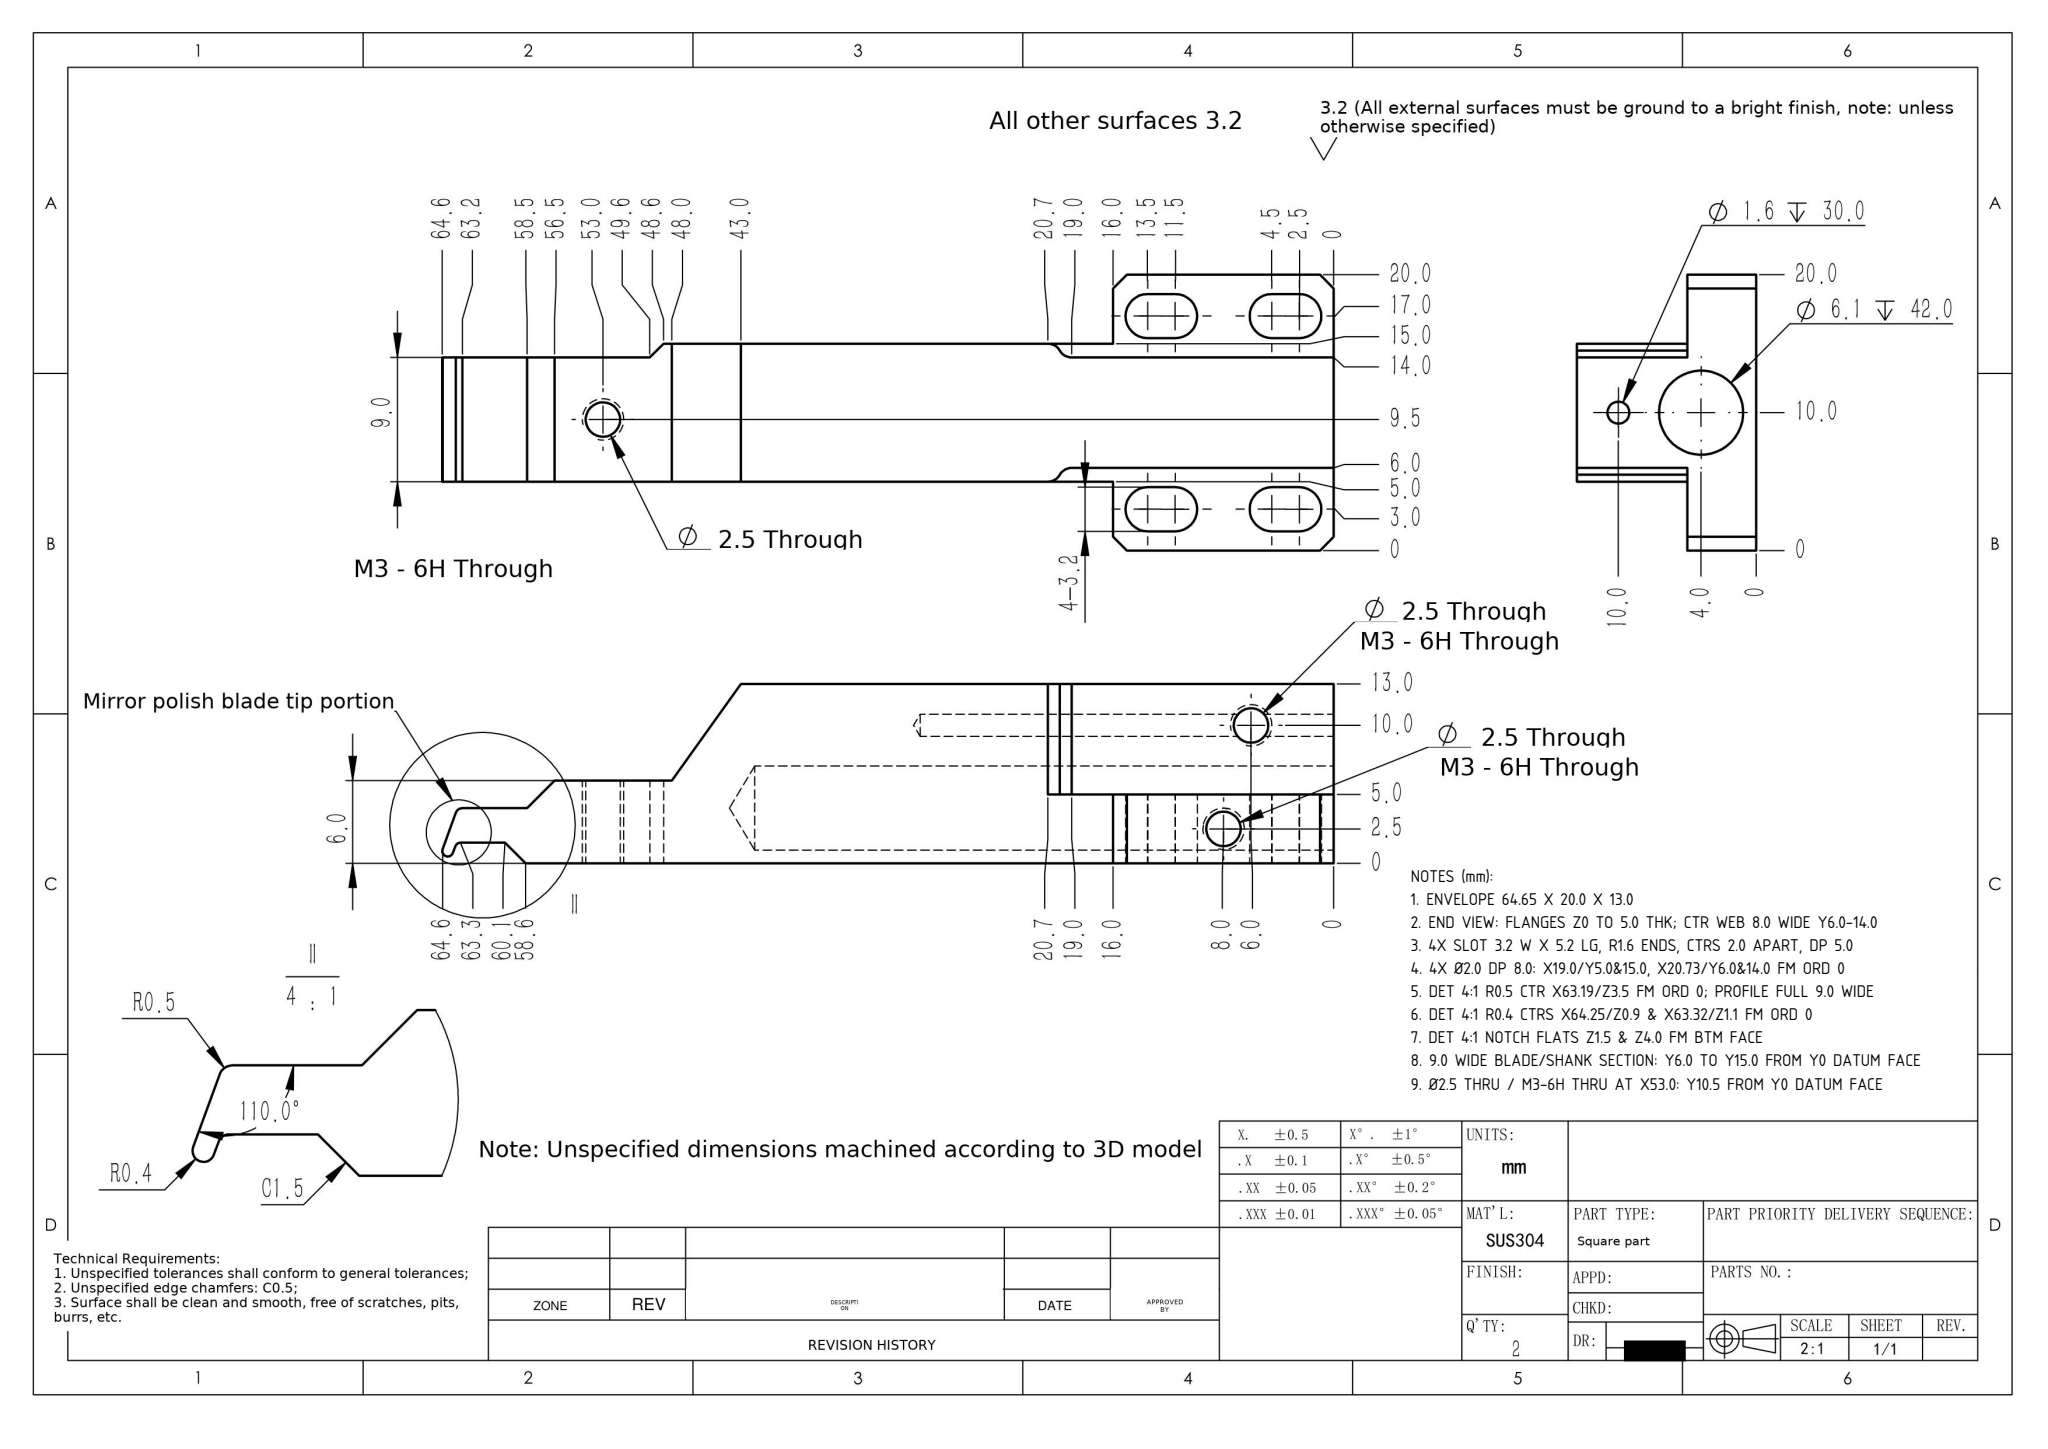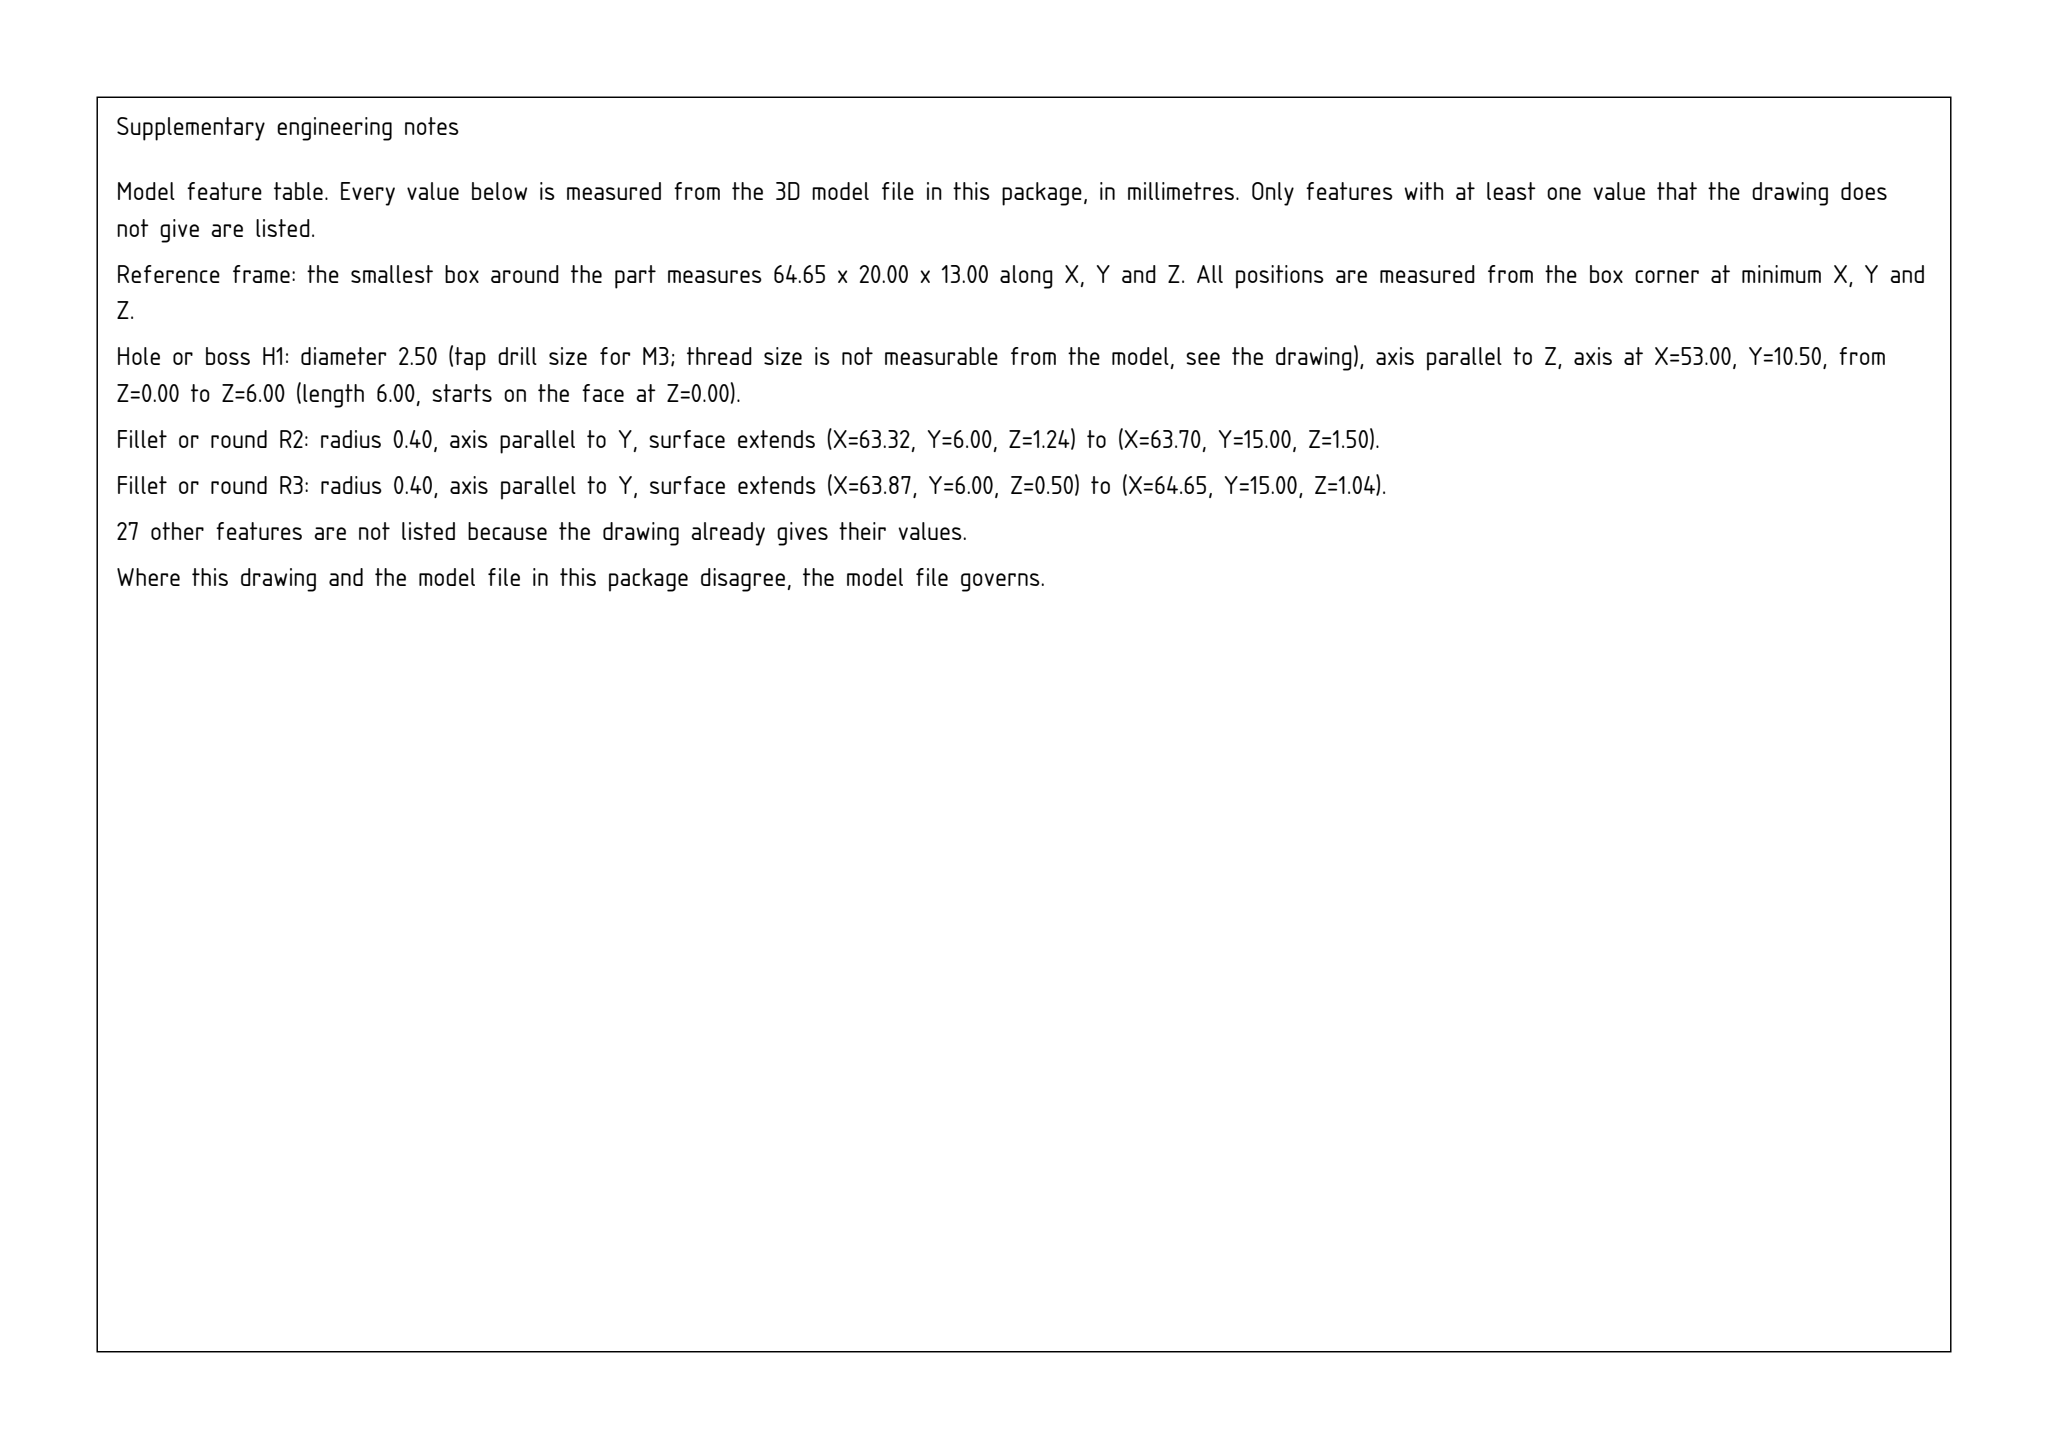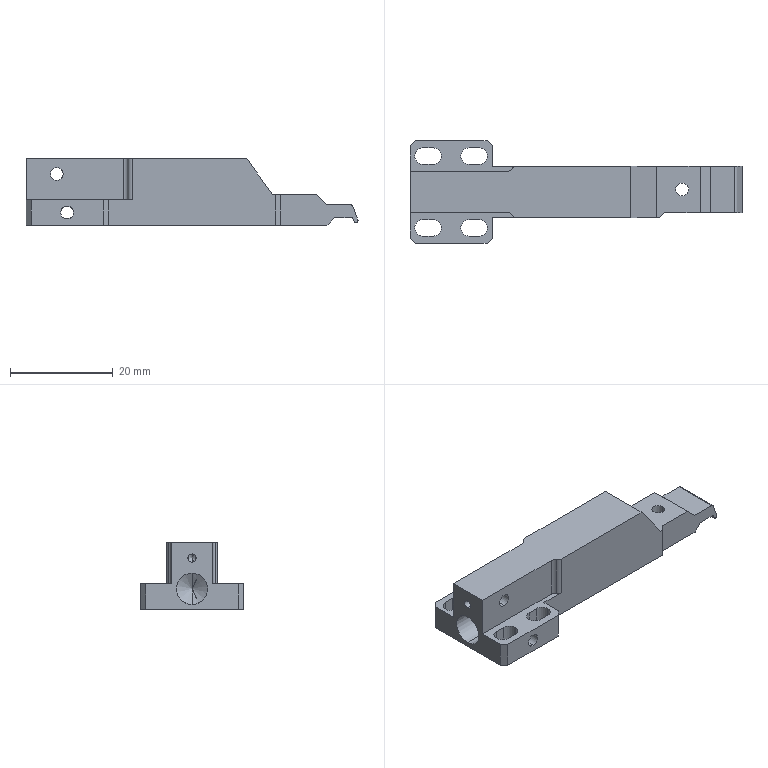Part | SolidWorks | mm | 1 solid | 74 faces | box 64.65 x 20 x 13 mm | volume 5503 mm3 | cylinder 35 | plane 35 | cone 4 | commonest cylinder face diameters 3.2 x12 2.5 x8 0.8 x4 1.6 x4 2 x4 6.1 x2 1 x1
Drawing notes:
ENVELOPE 64.65 X 20.0 X 13.0 | from the solid: bbox_xyz 64.646 x 20.0 x 13.0
END VIEW: FLANGES Z0 TO 5.0 THK; CTR WEB 8.0 WIDE Y6.0-14.0 | from the solid: z-planes 0/5.0; d2.5 y-hole len 8.0 betw y-planes 6.0 & 14.0
4X SLOT 3.2 W X 5.2 LG, R1.6 ENDS, CTRS 2.0 APART, DP 5.0 | from the solid: d3.2 z-cyls at x2.5/4.5 & x11.5/13.5, y3.0 & y17.0, len 5.0
4X Ø2.0 DP 8.0: X19.0/Y5.0&15.0, X20.73/Y6.0&14.0 FM ORD 0 | from the solid: dia 2.0 z-cyls len 8.0 at (19.0,5.0),(19.0,15.0),(20.73,6.0),(20.73,14.0)
DET 4:1 R0.5 CTR X63.19/Z3.5 FM ORD 0; PROFILE FULL 9.0 WIDE | from the solid: cyl d1.0 axis y at (63.19,z3.5), len 9.0 = shank width y5.0-14.0
DET 4:1 R0.4 CTRS X64.25/Z0.9 & X63.32/Z1.1 FM ORD 0 | from the solid: cyl d0.8 axis y at (63.32,z1.1) and (64.25,z0.9), len 9.0
DET 4:1 NOTCH FLATS Z1.5 & Z4.0 FM BTM FACE | from the solid: z-normal planes at 1.5 and 4.0 within blade tip zone
9.0 WIDE BLADE/SHANK SECTION: Y6.0 TO Y15.0 FROM Y0 DATUM FACE | from the solid: y planes at 6.0 and 15.0 bound the 9.0 band; bbox Y0-20.0
Ø2.5 THRU / M3-6H THRU AT X53.0: Y10.5 FROM Y0 DATUM FACE | from the solid: cylinder [2.5,'z',[53.0,10.5,null],6.0]